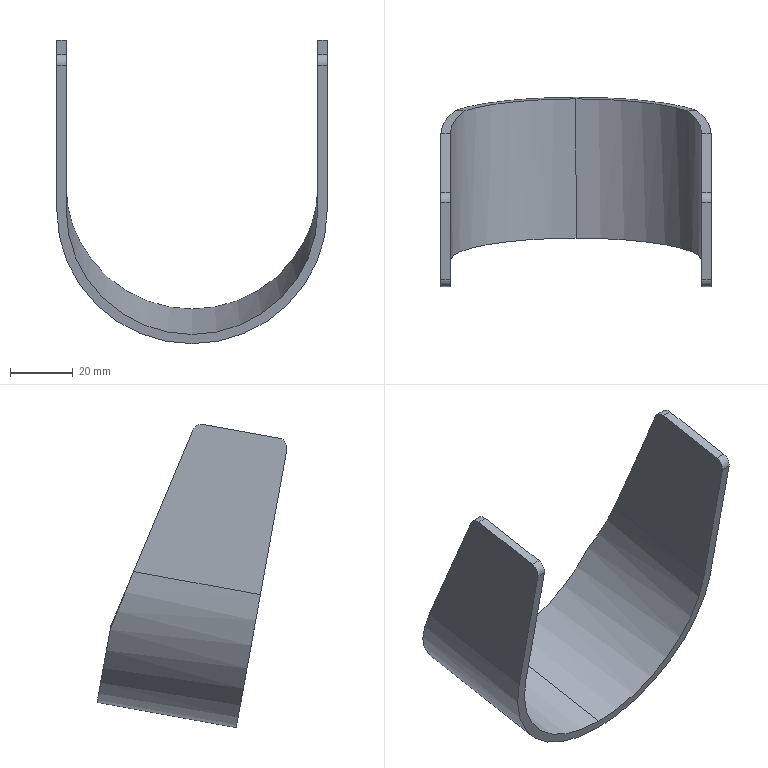Component | SolidWorks | ButtonStation-1_Two-HandButtonGuardRing-1 | 1 solid | 20 faces | box 86 x 60.42 x 96.48 mm | volume 28003 mm3 | plane 10 | cylinder 8 | spline 2 | commonest cylinder face diameters 6 x4 86 x2 80 x2 | material Plain Carbon Steel
STEP:
#1=COLOUR_RGB('',0.7922,0.8196,0.9333);
#2=FILL_AREA_STYLE_COLOUR('',#1);
#3=FILL_AREA_STYLE('',(#2));
#4=SURFACE_STYLE_FILL_AREA(#3);
#5=SURFACE_SIDE_STYLE('',(#4));
#6=SURFACE_STYLE_USAGE(.BOTH.,#5);
#7=PRESENTATION_STYLE_ASSIGNMENT((#6));
#8=CARTESIAN_POINT('',(-11.233,31.849,24.027));
#9=VERTEX_POINT('',#8);
#10=CARTESIAN_POINT('',(-9.724,32.014,23.118));
#11=VERTEX_POINT('',#10);
#12=CARTESIAN_POINT('',(-9.724,31.711,24.783));
#13=DIRECTION('',(0.,-0.9839,-0.1789));
#14=DIRECTION('',(0.,0.1789,-0.9839));
#15=AXIS2_PLACEMENT_3D('',#12,#13,#14);
#16=CIRCLE('',#15,1.693);
#17=EDGE_CURVE('',#9,#11,#16,.T.);
#18=ORIENTED_EDGE('',*,*,#17,.T.);
#19=CARTESIAN_POINT('',(-9.724,30.271,22.801));
#20=VERTEX_POINT('',#19);
#21=CARTESIAN_POINT('',(-9.724,32.014,23.118));
#22=DIRECTION('',(0.,-0.9839,-0.1789));
#23=VECTOR('',#22,39.37);
#24=LINE('',#21,#23);
#25=EDGE_CURVE('',#11,#20,#24,.T.);
#26=ORIENTED_EDGE('',*,*,#25,.T.);
#27=CARTESIAN_POINT('',(-11.417,29.968,24.466));
#28=VERTEX_POINT('',#27);
#29=CARTESIAN_POINT('',(-9.724,29.968,24.466));
#30=DIRECTION('',(-0.,0.9839,0.1789));
#31=DIRECTION('',(0.,0.1789,-0.9839));
#32=AXIS2_PLACEMENT_3D('',#29,#30,#31);
#33=CIRCLE('',#32,1.693);
#34=EDGE_CURVE('',#20,#28,#33,.T.);
#35=ORIENTED_EDGE('',*,*,#34,.T.);
#36=CARTESIAN_POINT('',(-11.417,31.556,24.755));
#37=VERTEX_POINT('',#36);
#38=CARTESIAN_POINT('',(-11.417,31.711,24.783));
#39=DIRECTION('',(-0.,0.9839,0.1789));
#40=VECTOR('',#39,39.37);
#41=LINE('',#38,#40);
#42=EDGE_CURVE('',#28,#37,#41,.T.);
#43=ORIENTED_EDGE('',*,*,#42,.T.);
#44=CARTESIAN_POINT('',(-11.417,31.556,24.755));
#45=CARTESIAN_POINT('',(-11.417,31.66,24.498));
#46=CARTESIAN_POINT('',(-11.353,31.759,24.251));
#47=CARTESIAN_POINT('',(-11.233,31.849,24.027));
#48=(BOUNDED_CURVE()B_SPLINE_CURVE(3,(#44,#45,#46,#47),.UNSPECIFIED.,.F.,.F.)B_SPLINE_CURVE_WITH_KNOTS((4,4),(0.,0.02054),.UNSPECIFIED.)CURVE()GEOMETRIC_REPRESENTATION_ITEM()RATIONAL_B_SPLINE_CURVE((0.5,0.5,0.5096,0.5288))REPRESENTATION_ITEM(''));
#49=EDGE_CURVE('',#37,#9,#48,.T.);
#50=ORIENTED_EDGE('',*,*,#49,.T.);
#51=EDGE_LOOP('',(#18,#26,#35,#43,#50));
#52=FACE_OUTER_BOUND('',#51,.T.);
#53=CARTESIAN_POINT('',(-9.724,31.711,24.783));
#54=DIRECTION('',(0.,-0.9839,-0.1789));
#55=DIRECTION('',(0.,0.1789,-0.9839));
#56=AXIS2_PLACEMENT_3D('',#53,#54,#55);
#57=CYLINDRICAL_SURFACE('',#56,1.693);
#58=ADVANCED_FACE('',(#52),#57,.T.);
#59=CARTESIAN_POINT('',(-9.724,31.993,23.234));
#60=VERTEX_POINT('',#59);
#61=CARTESIAN_POINT('',(-8.321,31.839,24.08));
#62=VERTEX_POINT('',#61);
#63=CARTESIAN_POINT('',(-9.724,31.711,24.783));
#64=DIRECTION('',(0.,-0.9839,-0.1789));
#65=DIRECTION('',(0.,0.1789,-0.9839));
#66=AXIS2_PLACEMENT_3D('',#63,#64,#65);
#67=CIRCLE('',#66,1.575);
#68=EDGE_CURVE('',#60,#62,#67,.T.);
#69=ORIENTED_EDGE('',*,*,#68,.F.);
#70=CARTESIAN_POINT('',(-9.724,30.25,22.917));
#71=VERTEX_POINT('',#70);
#72=CARTESIAN_POINT('',(-9.724,31.993,23.234));
#73=DIRECTION('',(0.,-0.9839,-0.1789));
#74=VECTOR('',#73,39.37);
#75=LINE('',#72,#74);
#76=EDGE_CURVE('',#60,#71,#75,.T.);
#77=ORIENTED_EDGE('',*,*,#76,.T.);
#78=CARTESIAN_POINT('',(-8.15,29.968,24.466));
#79=VERTEX_POINT('',#78);
#80=CARTESIAN_POINT('',(-9.724,29.968,24.466));
#81=DIRECTION('',(-0.,0.9839,0.1789));
#82=DIRECTION('',(0.,0.1789,-0.9839));
#83=AXIS2_PLACEMENT_3D('',#80,#81,#82);
#84=CIRCLE('',#83,1.575);
#85=EDGE_CURVE('',#79,#71,#84,.T.);
#86=ORIENTED_EDGE('',*,*,#85,.F.);
#87=CARTESIAN_POINT('',(-8.15,31.556,24.755));
#88=VERTEX_POINT('',#87);
#89=CARTESIAN_POINT('',(-8.15,31.711,24.783));
#90=DIRECTION('',(0.,-0.9839,-0.1789));
#91=VECTOR('',#90,39.37);
#92=LINE('',#89,#91);
#93=EDGE_CURVE('',#88,#79,#92,.T.);
#94=ORIENTED_EDGE('',*,*,#93,.F.);
#95=CARTESIAN_POINT('',(-8.321,31.839,24.08));
#96=CARTESIAN_POINT('',(-8.209,31.752,24.288));
#97=CARTESIAN_POINT('',(-8.15,31.656,24.517));
#98=CARTESIAN_POINT('',(-8.15,31.556,24.755));
#99=(BOUNDED_CURVE()B_SPLINE_CURVE(3,(#95,#96,#97,#98),.UNSPECIFIED.,.F.,.F.)B_SPLINE_CURVE_WITH_KNOTS((4,4),(0.,0.01915),.UNSPECIFIED.)CURVE()GEOMETRIC_REPRESENTATION_ITEM()RATIONAL_B_SPLINE_CURVE((0.5288,0.5096,0.5,0.5))REPRESENTATION_ITEM(''));
#100=EDGE_CURVE('',#62,#88,#99,.T.);
#101=ORIENTED_EDGE('',*,*,#100,.F.);
#102=EDGE_LOOP('',(#69,#77,#86,#94,#101));
#103=FACE_OUTER_BOUND('',#102,.T.);
#104=CARTESIAN_POINT('',(-9.724,31.711,24.783));
#105=DIRECTION('',(0.,-0.9839,-0.1789));
#106=DIRECTION('',(0.,0.1789,-0.9839));
#107=AXIS2_PLACEMENT_3D('',#104,#105,#106);
#108=CYLINDRICAL_SURFACE('',#107,1.575);
#109=ADVANCED_FACE('',(#103),#108,.F.);
#110=ORIENTED_EDGE('',*,*,#25,.F.);
#111=CARTESIAN_POINT('',(-8.216,31.849,24.027));
#112=VERTEX_POINT('',#111);
#113=CARTESIAN_POINT('',(-9.724,31.711,24.783));
#114=DIRECTION('',(0.,-0.9839,-0.1789));
#115=DIRECTION('',(0.,0.1789,-0.9839));
#116=AXIS2_PLACEMENT_3D('',#113,#114,#115);
#117=CIRCLE('',#116,1.693);
#118=EDGE_CURVE('',#11,#112,#117,.T.);
#119=ORIENTED_EDGE('',*,*,#118,.T.);
#120=CARTESIAN_POINT('',(-8.031,31.556,24.755));
#121=VERTEX_POINT('',#120);
#122=CARTESIAN_POINT('',(-8.216,31.849,24.027));
#123=CARTESIAN_POINT('',(-8.095,31.759,24.251));
#124=CARTESIAN_POINT('',(-8.031,31.66,24.498));
#125=CARTESIAN_POINT('',(-8.031,31.556,24.755));
#126=(BOUNDED_CURVE()B_SPLINE_CURVE(3,(#122,#123,#124,#125),.UNSPECIFIED.,.F.,.F.)B_SPLINE_CURVE_WITH_KNOTS((4,4),(0.,0.02054),.UNSPECIFIED.)CURVE()GEOMETRIC_REPRESENTATION_ITEM()RATIONAL_B_SPLINE_CURVE((0.5288,0.5096,0.5,0.5))REPRESENTATION_ITEM(''));
#127=EDGE_CURVE('',#112,#121,#126,.T.);
#128=ORIENTED_EDGE('',*,*,#127,.T.);
#129=CARTESIAN_POINT('',(-8.031,29.968,24.466));
#130=VERTEX_POINT('',#129);
#131=CARTESIAN_POINT('',(-8.031,31.711,24.783));
#132=DIRECTION('',(0.,-0.9839,-0.1789));
#133=VECTOR('',#132,39.37);
#134=LINE('',#131,#133);
#135=EDGE_CURVE('',#121,#130,#134,.T.);
#136=ORIENTED_EDGE('',*,*,#135,.T.);
#137=CARTESIAN_POINT('',(-9.724,29.968,24.466));
#138=DIRECTION('',(-0.,0.9839,0.1789));
#139=DIRECTION('',(0.,0.1789,-0.9839));
#140=AXIS2_PLACEMENT_3D('',#137,#138,#139);
#141=CIRCLE('',#140,1.693);
#142=EDGE_CURVE('',#130,#20,#141,.T.);
#143=ORIENTED_EDGE('',*,*,#142,.T.);
#144=EDGE_LOOP('',(#110,#119,#128,#136,#143));
#145=FACE_OUTER_BOUND('',#144,.T.);
#146=CARTESIAN_POINT('',(-9.724,31.711,24.783));
#147=DIRECTION('',(0.,-0.9839,-0.1789));
#148=DIRECTION('',(0.,0.1789,-0.9839));
#149=AXIS2_PLACEMENT_3D('',#146,#147,#148);
#150=CYLINDRICAL_SURFACE('',#149,1.693);
#151=ADVANCED_FACE('',(#145),#150,.T.);
#152=CARTESIAN_POINT('',(-11.417,29.637,26.287));
#153=VERTEX_POINT('',#152);
#154=CARTESIAN_POINT('',(-11.417,29.968,24.466));
#155=DIRECTION('',(-0.,-0.1789,0.9839));
#156=VECTOR('',#155,39.37);
#157=LINE('',#154,#156);
#158=EDGE_CURVE('',#28,#153,#157,.T.);
#159=ORIENTED_EDGE('',*,*,#158,.F.);
#160=ORIENTED_EDGE('',*,*,#34,.F.);
#161=ORIENTED_EDGE('',*,*,#142,.F.);
#162=CARTESIAN_POINT('',(-8.031,29.637,26.287));
#163=VERTEX_POINT('',#162);
#164=CARTESIAN_POINT('',(-8.031,29.968,24.466));
#165=DIRECTION('',(-0.,-0.1789,0.9839));
#166=VECTOR('',#165,39.37);
#167=LINE('',#164,#166);
#168=EDGE_CURVE('',#130,#163,#167,.T.);
#169=ORIENTED_EDGE('',*,*,#168,.T.);
#170=CARTESIAN_POINT('',(-8.15,29.637,26.287));
#171=VERTEX_POINT('',#170);
#172=CARTESIAN_POINT('',(-11.417,29.637,26.287));
#173=DIRECTION('',(-1.,-0.,-0.));
#174=VECTOR('',#173,39.37);
#175=LINE('',#172,#174);
#176=EDGE_CURVE('',#163,#171,#175,.T.);
#177=ORIENTED_EDGE('',*,*,#176,.T.);
#178=CARTESIAN_POINT('',(-8.15,29.968,24.466));
#179=DIRECTION('',(0.,0.1789,-0.9839));
#180=VECTOR('',#179,39.37);
#181=LINE('',#178,#180);
#182=EDGE_CURVE('',#171,#79,#181,.T.);
#183=ORIENTED_EDGE('',*,*,#182,.T.);
#184=ORIENTED_EDGE('',*,*,#85,.T.);
#185=CARTESIAN_POINT('',(-11.299,29.968,24.466));
#186=VERTEX_POINT('',#185);
#187=CARTESIAN_POINT('',(-9.724,29.968,24.466));
#188=DIRECTION('',(-0.,0.9839,0.1789));
#189=DIRECTION('',(0.,0.1789,-0.9839));
#190=AXIS2_PLACEMENT_3D('',#187,#188,#189);
#191=CIRCLE('',#190,1.575);
#192=EDGE_CURVE('',#71,#186,#191,.T.);
#193=ORIENTED_EDGE('',*,*,#192,.T.);
#194=CARTESIAN_POINT('',(-11.299,29.637,26.287));
#195=VERTEX_POINT('',#194);
#196=CARTESIAN_POINT('',(-11.299,29.968,24.466));
#197=DIRECTION('',(0.,0.1789,-0.9839));
#198=VECTOR('',#197,39.37);
#199=LINE('',#196,#198);
#200=EDGE_CURVE('',#195,#186,#199,.T.);
#201=ORIENTED_EDGE('',*,*,#200,.F.);
#202=CARTESIAN_POINT('',(-9.724,29.637,26.287));
#203=DIRECTION('',(1.,0.,0.));
#204=VECTOR('',#203,39.37);
#205=LINE('',#202,#204);
#206=EDGE_CURVE('',#153,#195,#205,.T.);
#207=ORIENTED_EDGE('',*,*,#206,.F.);
#208=EDGE_LOOP('',(#159,#160,#161,#169,#177,#183,#184,#193,#201,#207));
#209=FACE_OUTER_BOUND('',#208,.T.);
#210=CARTESIAN_POINT('',(-8.15,29.968,24.466));
#211=DIRECTION('',(0.,-0.9839,-0.1789));
#212=DIRECTION('',(0.,0.1789,-0.9839));
#213=AXIS2_PLACEMENT_3D('',#210,#211,#212);
#214=PLANE('',#213);
#215=ADVANCED_FACE('',(#209),#214,.T.);
#216=CARTESIAN_POINT('',(-8.031,30.685,26.597));
#217=VERTEX_POINT('',#216);
#218=CARTESIAN_POINT('',(-8.031,30.815,26.527));
#219=VERTEX_POINT('',#218);
#220=CARTESIAN_POINT('',(-8.031,30.706,26.481));
#221=DIRECTION('',(-1.,-0.,-0.));
#222=DIRECTION('',(0.,-0.9839,-0.1789));
#223=AXIS2_PLACEMENT_3D('',#220,#221,#222);
#224=CIRCLE('',#223,0.1181);
#225=EDGE_CURVE('',#217,#219,#224,.T.);
#226=ORIENTED_EDGE('',*,*,#225,.F.);
#227=CARTESIAN_POINT('',(-8.031,29.732,26.424));
#228=VERTEX_POINT('',#227);
#229=CARTESIAN_POINT('',(-8.031,31.359,26.72));
#230=DIRECTION('',(-0.,0.9839,0.1789));
#231=VECTOR('',#230,39.37);
#232=LINE('',#229,#231);
#233=EDGE_CURVE('',#228,#217,#232,.T.);
#234=ORIENTED_EDGE('',*,*,#233,.F.);
#235=CARTESIAN_POINT('',(-8.031,29.753,26.308));
#236=DIRECTION('',(-1.,-0.,-0.));
#237=DIRECTION('',(0.,-0.1789,0.9839));
#238=AXIS2_PLACEMENT_3D('',#235,#236,#237);
#239=CIRCLE('',#238,0.1181);
#240=EDGE_CURVE('',#163,#228,#239,.T.);
#241=ORIENTED_EDGE('',*,*,#240,.F.);
#242=ORIENTED_EDGE('',*,*,#168,.F.);
#243=ORIENTED_EDGE('',*,*,#135,.F.);
#244=CARTESIAN_POINT('',(-8.031,30.815,26.527));
#245=DIRECTION('',(-0.,0.3861,-0.9224));
#246=VECTOR('',#245,39.37);
#247=LINE('',#244,#246);
#248=EDGE_CURVE('',#219,#121,#247,.T.);
#249=ORIENTED_EDGE('',*,*,#248,.F.);
#250=EDGE_LOOP('',(#226,#234,#241,#242,#243,#249));
#251=FACE_OUTER_BOUND('',#250,.T.);
#252=CARTESIAN_POINT('',(-8.031,31.711,24.783));
#253=DIRECTION('',(-1.,-0.,-0.));
#254=DIRECTION('',(-0.,-0.1789,0.9839));
#255=AXIS2_PLACEMENT_3D('',#252,#253,#254);
#256=PLANE('',#255);
#257=ADVANCED_FACE('',(#251),#256,.F.);
#258=ORIENTED_EDGE('',*,*,#127,.F.);
#259=CARTESIAN_POINT('',(-8.269,31.844,24.053));
#260=DIRECTION('',(-0.8909,-0.08124,0.4468));
#261=VECTOR('',#260,39.37);
#262=LINE('',#259,#261);
#263=EDGE_CURVE('',#112,#62,#262,.T.);
#264=ORIENTED_EDGE('',*,*,#263,.T.);
#265=ORIENTED_EDGE('',*,*,#100,.T.);
#266=CARTESIAN_POINT('',(-8.091,31.556,24.755));
#267=DIRECTION('',(1.,0.,0.));
#268=VECTOR('',#267,39.37);
#269=LINE('',#266,#268);
#270=EDGE_CURVE('',#88,#121,#269,.T.);
#271=ORIENTED_EDGE('',*,*,#270,.T.);
#272=EDGE_LOOP('',(#258,#264,#265,#271));
#273=FACE_OUTER_BOUND('',#272,.T.);
#274=CARTESIAN_POINT('',(-9.724,30.934,26.242));
#275=CARTESIAN_POINT('',(-9.724,30.927,26.281));
#276=CARTESIAN_POINT('',(-9.724,30.92,26.32));
#277=CARTESIAN_POINT('',(-9.724,30.913,26.359));
#278=CARTESIAN_POINT('',(-12.874,30.934,26.242));
#279=CARTESIAN_POINT('',(-12.953,30.927,26.281));
#280=CARTESIAN_POINT('',(-13.031,30.92,26.32));
#281=CARTESIAN_POINT('',(-13.11,30.913,26.359));
#282=CARTESIAN_POINT('',(-12.874,32.179,23.268));
#283=CARTESIAN_POINT('',(-12.953,32.186,23.229));
#284=CARTESIAN_POINT('',(-13.031,32.193,23.19));
#285=CARTESIAN_POINT('',(-13.11,32.2,23.151));
#286=CARTESIAN_POINT('',(-9.724,32.179,23.268));
#287=CARTESIAN_POINT('',(-9.724,32.186,23.229));
#288=CARTESIAN_POINT('',(-9.724,32.193,23.19));
#289=CARTESIAN_POINT('',(-9.724,32.2,23.151));
#290=CARTESIAN_POINT('',(-6.575,32.179,23.268));
#291=CARTESIAN_POINT('',(-6.496,32.186,23.229));
#292=CARTESIAN_POINT('',(-6.417,32.193,23.19));
#293=CARTESIAN_POINT('',(-6.339,32.2,23.151));
#294=CARTESIAN_POINT('',(-6.575,30.934,26.242));
#295=CARTESIAN_POINT('',(-6.496,30.927,26.281));
#296=CARTESIAN_POINT('',(-6.417,30.92,26.32));
#297=CARTESIAN_POINT('',(-6.339,30.913,26.359));
#298=CARTESIAN_POINT('',(-9.724,30.934,26.242));
#299=CARTESIAN_POINT('',(-9.724,30.927,26.281));
#300=CARTESIAN_POINT('',(-9.724,30.92,26.32));
#301=CARTESIAN_POINT('',(-9.724,30.913,26.359));
#302=(BOUNDED_SURFACE()B_SPLINE_SURFACE(3,3,((#274,#275,#276,#277),(#278,#279,#280,#281),(#282,#283,#284,#285),(#286,#287,#288,#289),(#290,#291,#292,#293),(#294,#295,#296,#297),(#298,#299,#300,#301)),.UNSPECIFIED.,.T.,.F.,.F.)B_SPLINE_SURFACE_WITH_KNOTS((4,3,4),(4,4),(0.,0.5,1.),(0.,1.),.UNSPECIFIED.)GEOMETRIC_REPRESENTATION_ITEM()RATIONAL_B_SPLINE_SURFACE(((1.,1.,1.,1.),(0.3333,0.3333,0.3333,0.3333),(0.3333,0.3333,0.3333,0.3333),(1.,1.,1.,1.),(0.3333,0.3333,0.3333,0.3333),(0.3333,0.3333,0.3333,0.3333),(1.,1.,1.,1.)))REPRESENTATION_ITEM('')SURFACE());
#303=ADVANCED_FACE('',(#273),#302,.T.);
#304=CARTESIAN_POINT('',(-11.127,31.839,24.08));
#305=VERTEX_POINT('',#304);
#306=CARTESIAN_POINT('',(-11.233,31.849,24.027));
#307=DIRECTION('',(0.8909,-0.08124,0.4468));
#308=VECTOR('',#307,39.37);
#309=LINE('',#306,#308);
#310=EDGE_CURVE('',#9,#305,#309,.T.);
#311=ORIENTED_EDGE('',*,*,#310,.T.);
#312=CARTESIAN_POINT('',(-9.724,31.711,24.783));
#313=DIRECTION('',(0.,-0.9839,-0.1789));
#314=DIRECTION('',(0.,0.1789,-0.9839));
#315=AXIS2_PLACEMENT_3D('',#312,#313,#314);
#316=CIRCLE('',#315,1.575);
#317=EDGE_CURVE('',#305,#60,#316,.T.);
#318=ORIENTED_EDGE('',*,*,#317,.T.);
#319=ORIENTED_EDGE('',*,*,#68,.T.);
#320=ORIENTED_EDGE('',*,*,#263,.F.);
#321=ORIENTED_EDGE('',*,*,#118,.F.);
#322=ORIENTED_EDGE('',*,*,#17,.F.);
#323=EDGE_LOOP('',(#311,#318,#319,#320,#321,#322));
#324=FACE_OUTER_BOUND('',#323,.T.);
#325=CARTESIAN_POINT('',(-11.299,31.711,24.783));
#326=DIRECTION('',(-0.,0.9839,0.1789));
#327=DIRECTION('',(-0.,-0.1789,0.9839));
#328=AXIS2_PLACEMENT_3D('',#325,#326,#327);
#329=PLANE('',#328);
#330=ADVANCED_FACE('',(#324),#329,.T.);
#331=ORIENTED_EDGE('',*,*,#76,.F.);
#332=ORIENTED_EDGE('',*,*,#317,.F.);
#333=CARTESIAN_POINT('',(-11.299,31.556,24.755));
#334=VERTEX_POINT('',#333);
#335=CARTESIAN_POINT('',(-11.299,31.556,24.755));
#336=CARTESIAN_POINT('',(-11.299,31.656,24.517));
#337=CARTESIAN_POINT('',(-11.24,31.752,24.288));
#338=CARTESIAN_POINT('',(-11.127,31.839,24.08));
#339=(BOUNDED_CURVE()B_SPLINE_CURVE(3,(#335,#336,#337,#338),.UNSPECIFIED.,.F.,.F.)B_SPLINE_CURVE_WITH_KNOTS((4,4),(0.,0.01915),.UNSPECIFIED.)CURVE()GEOMETRIC_REPRESENTATION_ITEM()RATIONAL_B_SPLINE_CURVE((0.5,0.5,0.5096,0.5288))REPRESENTATION_ITEM(''));
#340=EDGE_CURVE('',#334,#305,#339,.T.);
#341=ORIENTED_EDGE('',*,*,#340,.F.);
#342=CARTESIAN_POINT('',(-11.299,31.711,24.783));
#343=DIRECTION('',(-0.,0.9839,0.1789));
#344=VECTOR('',#343,39.37);
#345=LINE('',#342,#344);
#346=EDGE_CURVE('',#186,#334,#345,.T.);
#347=ORIENTED_EDGE('',*,*,#346,.F.);
#348=ORIENTED_EDGE('',*,*,#192,.F.);
#349=EDGE_LOOP('',(#331,#332,#341,#347,#348));
#350=FACE_OUTER_BOUND('',#349,.T.);
#351=CARTESIAN_POINT('',(-9.724,31.711,24.783));
#352=DIRECTION('',(0.,-0.9839,-0.1789));
#353=DIRECTION('',(0.,0.1789,-0.9839));
#354=AXIS2_PLACEMENT_3D('',#351,#352,#353);
#355=CYLINDRICAL_SURFACE('',#354,1.575);
#356=ADVANCED_FACE('',(#350),#355,.F.);
#357=CARTESIAN_POINT('',(-8.15,30.815,26.527));
#358=VERTEX_POINT('',#357);
#359=CARTESIAN_POINT('',(-8.15,30.815,26.527));
#360=DIRECTION('',(-1.,-0.,-0.));
#361=VECTOR('',#360,39.37);
#362=LINE('',#359,#361);
#363=EDGE_CURVE('',#219,#358,#362,.T.);
#364=ORIENTED_EDGE('',*,*,#363,.F.);
#365=ORIENTED_EDGE('',*,*,#248,.T.);
#366=ORIENTED_EDGE('',*,*,#270,.F.);
#367=CARTESIAN_POINT('',(-8.15,31.569,24.724));
#368=DIRECTION('',(-0.,0.3861,-0.9224));
#369=VECTOR('',#368,39.37);
#370=LINE('',#367,#369);
#371=EDGE_CURVE('',#358,#88,#370,.T.);
#372=ORIENTED_EDGE('',*,*,#371,.F.);
#373=EDGE_LOOP('',(#364,#365,#366,#372));
#374=FACE_OUTER_BOUND('',#373,.T.);
#375=CARTESIAN_POINT('',(-8.15,31.569,24.724));
#376=DIRECTION('',(0.,-0.9224,-0.3861));
#377=DIRECTION('',(-0.,0.3861,-0.9224));
#378=AXIS2_PLACEMENT_3D('',#375,#376,#377);
#379=PLANE('',#378);
#380=ADVANCED_FACE('',(#374),#379,.F.);
#381=ORIENTED_EDGE('',*,*,#225,.T.);
#382=ORIENTED_EDGE('',*,*,#363,.T.);
#383=CARTESIAN_POINT('',(-8.15,30.685,26.597));
#384=VERTEX_POINT('',#383);
#385=CARTESIAN_POINT('',(-8.15,30.706,26.481));
#386=DIRECTION('',(1.,0.,0.));
#387=DIRECTION('',(0.,-0.9839,-0.1789));
#388=AXIS2_PLACEMENT_3D('',#385,#386,#387);
#389=CIRCLE('',#388,0.1181);
#390=EDGE_CURVE('',#358,#384,#389,.T.);
#391=ORIENTED_EDGE('',*,*,#390,.T.);
#392=CARTESIAN_POINT('',(-8.15,30.685,26.597));
#393=DIRECTION('',(1.,0.,0.));
#394=VECTOR('',#393,39.37);
#395=LINE('',#392,#394);
#396=EDGE_CURVE('',#384,#217,#395,.T.);
#397=ORIENTED_EDGE('',*,*,#396,.T.);
#398=EDGE_LOOP('',(#381,#382,#391,#397));
#399=FACE_OUTER_BOUND('',#398,.T.);
#400=CARTESIAN_POINT('',(-8.15,30.706,26.481));
#401=DIRECTION('',(-1.,-0.,-0.));
#402=DIRECTION('',(0.,-0.9839,-0.1789));
#403=AXIS2_PLACEMENT_3D('',#400,#401,#402);
#404=CYLINDRICAL_SURFACE('',#403,0.1181);
#405=ADVANCED_FACE('',(#399),#404,.T.);
#406=CARTESIAN_POINT('',(-8.15,29.732,26.424));
#407=VERTEX_POINT('',#406);
#408=CARTESIAN_POINT('',(-8.15,31.359,26.72));
#409=DIRECTION('',(0.,-0.9839,-0.1789));
#410=VECTOR('',#409,39.37);
#411=LINE('',#408,#410);
#412=EDGE_CURVE('',#384,#407,#411,.T.);
#413=ORIENTED_EDGE('',*,*,#412,.T.);
#414=CARTESIAN_POINT('',(-8.031,29.732,26.424));
#415=DIRECTION('',(1.,0.,0.));
#416=VECTOR('',#415,39.37);
#417=LINE('',#414,#416);
#418=EDGE_CURVE('',#407,#228,#417,.T.);
#419=ORIENTED_EDGE('',*,*,#418,.T.);
#420=ORIENTED_EDGE('',*,*,#233,.T.);
#421=ORIENTED_EDGE('',*,*,#396,.F.);
#422=EDGE_LOOP('',(#413,#419,#420,#421));
#423=FACE_OUTER_BOUND('',#422,.T.);
#424=CARTESIAN_POINT('',(-8.031,31.359,26.72));
#425=DIRECTION('',(-0.,-0.1789,0.9839));
#426=DIRECTION('',(1.,0.,0.));
#427=AXIS2_PLACEMENT_3D('',#424,#425,#426);
#428=PLANE('',#427);
#429=ADVANCED_FACE('',(#423),#428,.T.);
#430=CARTESIAN_POINT('',(-8.15,29.753,26.308));
#431=DIRECTION('',(1.,0.,0.));
#432=DIRECTION('',(0.,-0.1789,0.9839));
#433=AXIS2_PLACEMENT_3D('',#430,#431,#432);
#434=CIRCLE('',#433,0.1181);
#435=EDGE_CURVE('',#407,#171,#434,.T.);
#436=ORIENTED_EDGE('',*,*,#435,.T.);
#437=ORIENTED_EDGE('',*,*,#176,.F.);
#438=ORIENTED_EDGE('',*,*,#240,.T.);
#439=ORIENTED_EDGE('',*,*,#418,.F.);
#440=EDGE_LOOP('',(#436,#437,#438,#439));
#441=FACE_OUTER_BOUND('',#440,.T.);
#442=CARTESIAN_POINT('',(-11.417,29.753,26.308));
#443=DIRECTION('',(-1.,-0.,-0.));
#444=DIRECTION('',(0.,-0.1789,0.9839));
#445=AXIS2_PLACEMENT_3D('',#442,#443,#444);
#446=CYLINDRICAL_SURFACE('',#445,0.1181);
#447=ADVANCED_FACE('',(#441),#446,.T.);
#448=ORIENTED_EDGE('',*,*,#49,.F.);
#449=CARTESIAN_POINT('',(-11.358,31.556,24.755));
#450=DIRECTION('',(1.,0.,0.));
#451=VECTOR('',#450,39.37);
#452=LINE('',#449,#451);
#453=EDGE_CURVE('',#37,#334,#452,.T.);
#454=ORIENTED_EDGE('',*,*,#453,.T.);
#455=ORIENTED_EDGE('',*,*,#340,.T.);
#456=ORIENTED_EDGE('',*,*,#310,.F.);
#457=EDGE_LOOP('',(#448,#454,#455,#456));
#458=FACE_OUTER_BOUND('',#457,.T.);
#459=CARTESIAN_POINT('',(-9.724,30.934,26.242));
#460=CARTESIAN_POINT('',(-9.724,30.927,26.281));
#461=CARTESIAN_POINT('',(-9.724,30.92,26.32));
#462=CARTESIAN_POINT('',(-9.724,30.913,26.359));
#463=CARTESIAN_POINT('',(-12.874,30.934,26.242));
#464=CARTESIAN_POINT('',(-12.953,30.927,26.281));
#465=CARTESIAN_POINT('',(-13.031,30.92,26.32));
#466=CARTESIAN_POINT('',(-13.11,30.913,26.359));
#467=CARTESIAN_POINT('',(-12.874,32.179,23.268));
#468=CARTESIAN_POINT('',(-12.953,32.186,23.229));
#469=CARTESIAN_POINT('',(-13.031,32.193,23.19));
#470=CARTESIAN_POINT('',(-13.11,32.2,23.151));
#471=CARTESIAN_POINT('',(-9.724,32.179,23.268));
#472=CARTESIAN_POINT('',(-9.724,32.186,23.229));
#473=CARTESIAN_POINT('',(-9.724,32.193,23.19));
#474=CARTESIAN_POINT('',(-9.724,32.2,23.151));
#475=CARTESIAN_POINT('',(-6.575,32.179,23.268));
#476=CARTESIAN_POINT('',(-6.496,32.186,23.229));
#477=CARTESIAN_POINT('',(-6.417,32.193,23.19));
#478=CARTESIAN_POINT('',(-6.339,32.2,23.151));
#479=CARTESIAN_POINT('',(-6.575,30.934,26.242));
#480=CARTESIAN_POINT('',(-6.496,30.927,26.281));
#481=CARTESIAN_POINT('',(-6.417,30.92,26.32));
#482=CARTESIAN_POINT('',(-6.339,30.913,26.359));
#483=CARTESIAN_POINT('',(-9.724,30.934,26.242));
#484=CARTESIAN_POINT('',(-9.724,30.927,26.281));
#485=CARTESIAN_POINT('',(-9.724,30.92,26.32));
#486=CARTESIAN_POINT('',(-9.724,30.913,26.359));
#487=(BOUNDED_SURFACE()B_SPLINE_SURFACE(3,3,((#459,#460,#461,#462),(#463,#464,#465,#466),(#467,#468,#469,#470),(#471,#472,#473,#474),(#475,#476,#477,#478),(#479,#480,#481,#482),(#483,#484,#485,#486)),.UNSPECIFIED.,.T.,.F.,.F.)B_SPLINE_SURFACE_WITH_KNOTS((4,3,4),(4,4),(0.,0.5,1.),(0.,1.),.UNSPECIFIED.)GEOMETRIC_REPRESENTATION_ITEM()RATIONAL_B_SPLINE_SURFACE(((1.,1.,1.,1.),(0.3333,0.3333,0.3333,0.3333),(0.3333,0.3333,0.3333,0.3333),(1.,1.,1.,1.),(0.3333,0.3333,0.3333,0.3333),(0.3333,0.3333,0.3333,0.3333),(1.,1.,1.,1.)))REPRESENTATION_ITEM('')SURFACE());
#488=ADVANCED_FACE('',(#458),#487,.T.);
#489=CARTESIAN_POINT('',(-11.417,30.815,26.527));
#490=VERTEX_POINT('',#489);
#491=CARTESIAN_POINT('',(-11.417,30.685,26.597));
#492=VERTEX_POINT('',#491);
#493=CARTESIAN_POINT('',(-11.417,30.706,26.481));
#494=DIRECTION('',(1.,0.,0.));
#495=DIRECTION('',(0.,0.1789,-0.9839));
#496=AXIS2_PLACEMENT_3D('',#493,#494,#495);
#497=CIRCLE('',#496,0.1181);
#498=EDGE_CURVE('',#490,#492,#497,.T.);
#499=ORIENTED_EDGE('',*,*,#498,.F.);
#500=CARTESIAN_POINT('',(-11.417,31.556,24.755));
#501=DIRECTION('',(0.,-0.3861,0.9224));
#502=VECTOR('',#501,39.37);
#503=LINE('',#500,#502);
#504=EDGE_CURVE('',#37,#490,#503,.T.);
#505=ORIENTED_EDGE('',*,*,#504,.F.);
#506=ORIENTED_EDGE('',*,*,#42,.F.);
#507=ORIENTED_EDGE('',*,*,#158,.T.);
#508=CARTESIAN_POINT('',(-11.417,29.732,26.424));
#509=VERTEX_POINT('',#508);
#510=CARTESIAN_POINT('',(-11.417,29.753,26.308));
#511=DIRECTION('',(1.,0.,0.));
#512=DIRECTION('',(0.,0.1789,-0.9839));
#513=AXIS2_PLACEMENT_3D('',#510,#511,#512);
#514=CIRCLE('',#513,0.1181);
#515=EDGE_CURVE('',#509,#153,#514,.T.);
#516=ORIENTED_EDGE('',*,*,#515,.F.);
#517=CARTESIAN_POINT('',(-11.417,31.359,26.72));
#518=DIRECTION('',(0.,-0.9839,-0.1789));
#519=VECTOR('',#518,39.37);
#520=LINE('',#517,#519);
#521=EDGE_CURVE('',#492,#509,#520,.T.);
#522=ORIENTED_EDGE('',*,*,#521,.F.);
#523=EDGE_LOOP('',(#499,#505,#506,#507,#516,#522));
#524=FACE_OUTER_BOUND('',#523,.T.);
#525=CARTESIAN_POINT('',(-11.417,31.711,24.783));
#526=DIRECTION('',(1.,0.,0.));
#527=DIRECTION('',(0.,0.1789,-0.9839));
#528=AXIS2_PLACEMENT_3D('',#525,#526,#527);
#529=PLANE('',#528);
#530=ADVANCED_FACE('',(#524),#529,.F.);
#531=ORIENTED_EDGE('',*,*,#200,.T.);
#532=ORIENTED_EDGE('',*,*,#346,.T.);
#533=CARTESIAN_POINT('',(-11.299,30.815,26.527));
#534=VERTEX_POINT('',#533);
#535=CARTESIAN_POINT('',(-11.299,31.556,24.755));
#536=DIRECTION('',(0.,-0.3861,0.9224));
#537=VECTOR('',#536,39.37);
#538=LINE('',#535,#537);
#539=EDGE_CURVE('',#334,#534,#538,.T.);
#540=ORIENTED_EDGE('',*,*,#539,.T.);
#541=CARTESIAN_POINT('',(-11.299,30.685,26.597));
#542=VERTEX_POINT('',#541);
#543=CARTESIAN_POINT('',(-11.299,30.706,26.481));
#544=DIRECTION('',(1.,0.,0.));
#545=DIRECTION('',(0.,0.1789,-0.9839));
#546=AXIS2_PLACEMENT_3D('',#543,#544,#545);
#547=CIRCLE('',#546,0.1181);
#548=EDGE_CURVE('',#534,#542,#547,.T.);
#549=ORIENTED_EDGE('',*,*,#548,.T.);
#550=CARTESIAN_POINT('',(-11.299,29.732,26.424));
#551=VERTEX_POINT('',#550);
#552=CARTESIAN_POINT('',(-11.299,31.359,26.72));
#553=DIRECTION('',(0.,-0.9839,-0.1789));
#554=VECTOR('',#553,39.37);
#555=LINE('',#552,#554);
#556=EDGE_CURVE('',#542,#551,#555,.T.);
#557=ORIENTED_EDGE('',*,*,#556,.T.);
#558=CARTESIAN_POINT('',(-11.299,29.753,26.308));
#559=DIRECTION('',(1.,0.,0.));
#560=DIRECTION('',(0.,0.1789,-0.9839));
#561=AXIS2_PLACEMENT_3D('',#558,#559,#560);
#562=CIRCLE('',#561,0.1181);
#563=EDGE_CURVE('',#551,#195,#562,.T.);
#564=ORIENTED_EDGE('',*,*,#563,.T.);
#565=EDGE_LOOP('',(#531,#532,#540,#549,#557,#564));
#566=FACE_OUTER_BOUND('',#565,.T.);
#567=CARTESIAN_POINT('',(-11.299,31.711,24.783));
#568=DIRECTION('',(1.,0.,0.));
#569=DIRECTION('',(0.,0.1789,-0.9839));
#570=AXIS2_PLACEMENT_3D('',#567,#568,#569);
#571=PLANE('',#570);
#572=ADVANCED_FACE('',(#566),#571,.T.);
#573=ORIENTED_EDGE('',*,*,#515,.T.);
#574=ORIENTED_EDGE('',*,*,#206,.T.);
#575=ORIENTED_EDGE('',*,*,#563,.F.);
#576=CARTESIAN_POINT('',(-9.724,29.732,26.424));
#577=DIRECTION('',(-1.,-0.,-0.));
#578=VECTOR('',#577,39.37);
#579=LINE('',#576,#578);
#580=EDGE_CURVE('',#551,#509,#579,.T.);
#581=ORIENTED_EDGE('',*,*,#580,.T.);
#582=EDGE_LOOP('',(#573,#574,#575,#581));
#583=FACE_OUTER_BOUND('',#582,.T.);
#584=CARTESIAN_POINT('',(-9.724,29.753,26.308));
#585=DIRECTION('',(1.,0.,0.));
#586=DIRECTION('',(0.,0.1789,-0.9839));
#587=AXIS2_PLACEMENT_3D('',#584,#585,#586);
#588=CYLINDRICAL_SURFACE('',#587,0.1181);
#589=ADVANCED_FACE('',(#583),#588,.T.);
#590=ORIENTED_EDGE('',*,*,#182,.F.);
#591=ORIENTED_EDGE('',*,*,#435,.F.);
#592=ORIENTED_EDGE('',*,*,#412,.F.);
#593=ORIENTED_EDGE('',*,*,#390,.F.);
#594=ORIENTED_EDGE('',*,*,#371,.T.);
#595=ORIENTED_EDGE('',*,*,#93,.T.);
#596=EDGE_LOOP('',(#590,#591,#592,#593,#594,#595));
#597=FACE_OUTER_BOUND('',#596,.T.);
#598=CARTESIAN_POINT('',(-8.15,31.711,24.783));
#599=DIRECTION('',(-1.,-0.,-0.));
#600=DIRECTION('',(-0.,-0.1789,0.9839));
#601=AXIS2_PLACEMENT_3D('',#598,#599,#600);
#602=PLANE('',#601);
#603=ADVANCED_FACE('',(#597),#602,.T.);
#604=CARTESIAN_POINT('',(-11.299,30.815,26.527));
#605=DIRECTION('',(-1.,-0.,-0.));
#606=VECTOR('',#605,39.37);
#607=LINE('',#604,#606);
#608=EDGE_CURVE('',#534,#490,#607,.T.);
#609=ORIENTED_EDGE('',*,*,#608,.F.);
#610=ORIENTED_EDGE('',*,*,#539,.F.);
#611=ORIENTED_EDGE('',*,*,#453,.F.);
#612=ORIENTED_EDGE('',*,*,#504,.T.);
#613=EDGE_LOOP('',(#609,#610,#611,#612));
#614=FACE_OUTER_BOUND('',#613,.T.);
#615=CARTESIAN_POINT('',(-11.299,31.569,24.724));
#616=DIRECTION('',(0.,-0.9224,-0.3861));
#617=DIRECTION('',(-0.,0.3861,-0.9224));
#618=AXIS2_PLACEMENT_3D('',#615,#616,#617);
#619=PLANE('',#618);
#620=ADVANCED_FACE('',(#614),#619,.F.);
#621=ORIENTED_EDGE('',*,*,#521,.T.);
#622=ORIENTED_EDGE('',*,*,#580,.F.);
#623=ORIENTED_EDGE('',*,*,#556,.F.);
#624=CARTESIAN_POINT('',(-11.299,30.685,26.597));
#625=DIRECTION('',(-1.,-0.,-0.));
#626=VECTOR('',#625,39.37);
#627=LINE('',#624,#626);
#628=EDGE_CURVE('',#542,#492,#627,.T.);
#629=ORIENTED_EDGE('',*,*,#628,.T.);
#630=EDGE_LOOP('',(#621,#622,#623,#629));
#631=FACE_OUTER_BOUND('',#630,.T.);
#632=CARTESIAN_POINT('',(-11.299,31.359,26.72));
#633=DIRECTION('',(-0.,-0.1789,0.9839));
#634=DIRECTION('',(1.,0.,0.));
#635=AXIS2_PLACEMENT_3D('',#632,#633,#634);
#636=PLANE('',#635);
#637=ADVANCED_FACE('',(#631),#636,.T.);
#638=ORIENTED_EDGE('',*,*,#498,.T.);
#639=ORIENTED_EDGE('',*,*,#628,.F.);
#640=ORIENTED_EDGE('',*,*,#548,.F.);
#641=ORIENTED_EDGE('',*,*,#608,.T.);
#642=EDGE_LOOP('',(#638,#639,#640,#641));
#643=FACE_OUTER_BOUND('',#642,.T.);
#644=CARTESIAN_POINT('',(-11.299,30.706,26.481));
#645=DIRECTION('',(1.,0.,0.));
#646=DIRECTION('',(0.,0.1789,-0.9839));
#647=AXIS2_PLACEMENT_3D('',#644,#645,#646);
#648=CYLINDRICAL_SURFACE('',#647,0.1181);
#649=ADVANCED_FACE('',(#643),#648,.T.);
#650=CLOSED_SHELL('',(#58,#109,#151,#215,#257,#303,#330,#356,#380,#405,#429,#447,#488,#530,#572,#589,#603,#620,#637,#649));
#651=MANIFOLD_SOLID_BREP('',#650);
#652=STYLED_ITEM('',(#7),#651);
#653=(LENGTH_UNIT()NAMED_UNIT(*)SI_UNIT($,.METRE.));
#654=LENGTH_MEASURE_WITH_UNIT(LENGTH_MEASURE(0.0254),#653);
#655=DIMENSIONAL_EXPONENTS(1.,0.,0.,0.,0.,0.,0.);
#656=(CONVERSION_BASED_UNIT('',#654)LENGTH_UNIT()NAMED_UNIT(#655));
#657=UNCERTAINTY_MEASURE_WITH_UNIT(LENGTH_MEASURE(0.00001),#656,'','');
#658=(NAMED_UNIT(*)PLANE_ANGLE_UNIT()SI_UNIT($,.RADIAN.));
#659=(NAMED_UNIT(*)SI_UNIT($,.STERADIAN.)SOLID_ANGLE_UNIT());
#660=(GEOMETRIC_REPRESENTATION_CONTEXT(3)GLOBAL_UNCERTAINTY_ASSIGNED_CONTEXT((#657))GLOBAL_UNIT_ASSIGNED_CONTEXT((#656,#658,#659))REPRESENTATION_CONTEXT('',''));
#661=MECHANICAL_DESIGN_GEOMETRIC_PRESENTATION_REPRESENTATION('',(#652),#660);
#662=PRESENTATION_LAYER_ASSIGNMENT('','',(#652));
#663=CARTESIAN_POINT('',(0.,0.,0.));
#664=DIRECTION('',(0.,0.,1.));
#665=DIRECTION('',(1.,0.,0.));
#666=AXIS2_PLACEMENT_3D('',#663,#664,#665);
#667=(LENGTH_UNIT()NAMED_UNIT(*)SI_UNIT($,.METRE.));
#668=LENGTH_MEASURE_WITH_UNIT(LENGTH_MEASURE(0.0254),#667);
#669=DIMENSIONAL_EXPONENTS(1.,0.,0.,0.,0.,0.,0.);
#670=(CONVERSION_BASED_UNIT('',#668)LENGTH_UNIT()NAMED_UNIT(#669));
#671=UNCERTAINTY_MEASURE_WITH_UNIT(LENGTH_MEASURE(0.00001),#670,'','');
#672=(NAMED_UNIT(*)PLANE_ANGLE_UNIT()SI_UNIT($,.RADIAN.));
#673=(NAMED_UNIT(*)SI_UNIT($,.STERADIAN.)SOLID_ANGLE_UNIT());
#674=(GEOMETRIC_REPRESENTATION_CONTEXT(3)GLOBAL_UNCERTAINTY_ASSIGNED_CONTEXT((#671))GLOBAL_UNIT_ASSIGNED_CONTEXT((#670,#672,#673))REPRESENTATION_CONTEXT('',''));
#675=ADVANCED_BREP_SHAPE_REPRESENTATION('',(#651,#666),#674);